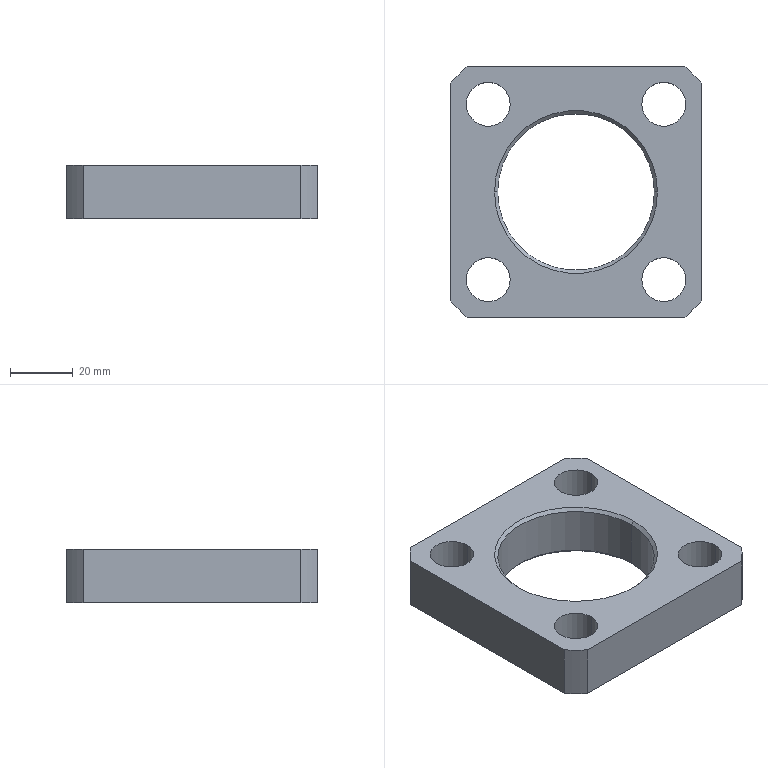Component | SolidWorks | Cylinder-1_Gland-1 | 1 solid | 24 faces | box 80 x 80 x 17 mm | volume 63907 mm3 | cylinder 14 | plane 6 | cone 4 | commonest cylinder face diameters 14 x8 106 x4 50 x2
STEP:
#1=CARTESIAN_POINT('',(-8.093,1.04,-7.612));
#2=VERTEX_POINT('',#1);
#3=CARTESIAN_POINT('',(-6.124,1.04,-7.612));
#4=VERTEX_POINT('',#3);
#5=CARTESIAN_POINT('',(-7.109,1.04,-7.612));
#6=DIRECTION('',(0.,-0.,-1.));
#7=DIRECTION('',(-1.,0.,0.));
#8=AXIS2_PLACEMENT_3D('',#5,#6,#7);
#9=CIRCLE('',#8,0.9843);
#10=EDGE_CURVE('',#2,#4,#9,.T.);
#11=ORIENTED_EDGE('',*,*,#10,.F.);
#12=CARTESIAN_POINT('',(-8.132,1.04,-7.652));
#13=VERTEX_POINT('',#12);
#14=CARTESIAN_POINT('',(-8.093,1.04,-7.612));
#15=DIRECTION('',(-0.7071,-0.,-0.7071));
#16=VECTOR('',#15,39.37);
#17=LINE('',#14,#16);
#18=EDGE_CURVE('',#2,#13,#17,.T.);
#19=ORIENTED_EDGE('',*,*,#18,.T.);
#20=CARTESIAN_POINT('',(-6.085,1.04,-7.652));
#21=VERTEX_POINT('',#20);
#22=CARTESIAN_POINT('',(-7.109,1.04,-7.652));
#23=DIRECTION('',(-0.,0.,1.));
#24=DIRECTION('',(-1.,0.,0.));
#25=AXIS2_PLACEMENT_3D('',#22,#23,#24);
#26=CIRCLE('',#25,1.024);
#27=EDGE_CURVE('',#21,#13,#26,.T.);
#28=ORIENTED_EDGE('',*,*,#27,.F.);
#29=CARTESIAN_POINT('',(-6.124,1.04,-7.612));
#30=DIRECTION('',(0.7071,-0.,-0.7071));
#31=VECTOR('',#30,39.37);
#32=LINE('',#29,#31);
#33=EDGE_CURVE('',#4,#21,#32,.T.);
#34=ORIENTED_EDGE('',*,*,#33,.F.);
#35=EDGE_LOOP('',(#11,#19,#28,#34));
#36=FACE_OUTER_BOUND('',#35,.T.);
#37=CARTESIAN_POINT('',(-7.109,1.04,-7.612));
#38=DIRECTION('',(0.,-0.,-1.));
#39=DIRECTION('',(1.,-0.,0.));
#40=AXIS2_PLACEMENT_3D('',#37,#38,#39);
#41=CONICAL_SURFACE('',#40,0.9843,0.7854);
#42=ADVANCED_FACE('',(#36),#41,.F.);
#43=CARTESIAN_POINT('',(-6.124,1.04,-7.022));
#44=VERTEX_POINT('',#43);
#45=CARTESIAN_POINT('',(-8.093,1.04,-7.022));
#46=VERTEX_POINT('',#45);
#47=CARTESIAN_POINT('',(-7.109,1.04,-7.022));
#48=DIRECTION('',(-0.,0.,1.));
#49=DIRECTION('',(-1.,0.,0.));
#50=AXIS2_PLACEMENT_3D('',#47,#48,#49);
#51=CIRCLE('',#50,0.9843);
#52=EDGE_CURVE('',#44,#46,#51,.T.);
#53=ORIENTED_EDGE('',*,*,#52,.F.);
#54=CARTESIAN_POINT('',(-6.085,1.04,-6.982));
#55=VERTEX_POINT('',#54);
#56=CARTESIAN_POINT('',(-6.085,1.04,-6.982));
#57=DIRECTION('',(0.7071,-0.,0.7071));
#58=VECTOR('',#57,39.37);
#59=LINE('',#56,#58);
#60=EDGE_CURVE('',#44,#55,#59,.T.);
#61=ORIENTED_EDGE('',*,*,#60,.T.);
#62=CARTESIAN_POINT('',(-8.132,1.04,-6.982));
#63=VERTEX_POINT('',#62);
#64=CARTESIAN_POINT('',(-7.109,1.04,-6.982));
#65=DIRECTION('',(0.,-0.,-1.));
#66=DIRECTION('',(-1.,0.,0.));
#67=AXIS2_PLACEMENT_3D('',#64,#65,#66);
#68=CIRCLE('',#67,1.024);
#69=EDGE_CURVE('',#63,#55,#68,.T.);
#70=ORIENTED_EDGE('',*,*,#69,.F.);
#71=CARTESIAN_POINT('',(-8.132,1.04,-6.982));
#72=DIRECTION('',(-0.7071,0.,0.7071));
#73=VECTOR('',#72,39.37);
#74=LINE('',#71,#73);
#75=EDGE_CURVE('',#46,#63,#74,.T.);
#76=ORIENTED_EDGE('',*,*,#75,.F.);
#77=EDGE_LOOP('',(#53,#61,#70,#76));
#78=FACE_OUTER_BOUND('',#77,.T.);
#79=CARTESIAN_POINT('',(-7.109,1.04,-6.982));
#80=DIRECTION('',(-0.,0.,1.));
#81=DIRECTION('',(-1.,0.,0.));
#82=AXIS2_PLACEMENT_3D('',#79,#80,#81);
#83=CONICAL_SURFACE('',#82,1.024,0.7854);
#84=ADVANCED_FACE('',(#78),#83,.F.);
#85=ORIENTED_EDGE('',*,*,#52,.T.);
#86=CARTESIAN_POINT('',(-8.093,1.04,-6.982));
#87=DIRECTION('',(0.,-0.,-1.));
#88=VECTOR('',#87,39.37);
#89=LINE('',#86,#88);
#90=EDGE_CURVE('',#46,#2,#89,.T.);
#91=ORIENTED_EDGE('',*,*,#90,.T.);
#92=ORIENTED_EDGE('',*,*,#10,.T.);
#93=CARTESIAN_POINT('',(-6.124,1.04,-6.982));
#94=DIRECTION('',(0.,-0.,-1.));
#95=VECTOR('',#94,39.37);
#96=LINE('',#93,#95);
#97=EDGE_CURVE('',#44,#4,#96,.T.);
#98=ORIENTED_EDGE('',*,*,#97,.F.);
#99=EDGE_LOOP('',(#85,#91,#92,#98));
#100=FACE_OUTER_BOUND('',#99,.T.);
#101=CARTESIAN_POINT('',(-7.109,1.04,-6.982));
#102=DIRECTION('',(0.,-0.,-1.));
#103=DIRECTION('',(1.,-0.,0.));
#104=AXIS2_PLACEMENT_3D('',#101,#102,#103);
#105=CYLINDRICAL_SURFACE('',#104,0.9843);
#106=ADVANCED_FACE('',(#100),#105,.F.);
#107=CARTESIAN_POINT('',(-8.486,2.142,-6.982));
#108=VERTEX_POINT('',#107);
#109=CARTESIAN_POINT('',(-7.935,2.142,-6.982));
#110=VERTEX_POINT('',#109);
#111=CARTESIAN_POINT('',(-8.211,2.142,-6.982));
#112=DIRECTION('',(0.,-0.,-1.));
#113=DIRECTION('',(-1.,0.,0.));
#114=AXIS2_PLACEMENT_3D('',#111,#112,#113);
#115=CIRCLE('',#114,0.2756);
#116=EDGE_CURVE('',#108,#110,#115,.T.);
#117=ORIENTED_EDGE('',*,*,#116,.F.);
#118=CARTESIAN_POINT('',(-8.486,2.142,-7.652));
#119=VERTEX_POINT('',#118);
#120=CARTESIAN_POINT('',(-8.486,2.142,-6.982));
#121=DIRECTION('',(0.,-0.,-1.));
#122=VECTOR('',#121,39.37);
#123=LINE('',#120,#122);
#124=EDGE_CURVE('',#108,#119,#123,.T.);
#125=ORIENTED_EDGE('',*,*,#124,.T.);
#126=CARTESIAN_POINT('',(-7.935,2.142,-7.652));
#127=VERTEX_POINT('',#126);
#128=CARTESIAN_POINT('',(-8.211,2.142,-7.652));
#129=DIRECTION('',(0.,-0.,-1.));
#130=DIRECTION('',(-1.,0.,0.));
#131=AXIS2_PLACEMENT_3D('',#128,#129,#130);
#132=CIRCLE('',#131,0.2756);
#133=EDGE_CURVE('',#119,#127,#132,.T.);
#134=ORIENTED_EDGE('',*,*,#133,.T.);
#135=CARTESIAN_POINT('',(-7.935,2.142,-6.982));
#136=DIRECTION('',(0.,-0.,-1.));
#137=VECTOR('',#136,39.37);
#138=LINE('',#135,#137);
#139=EDGE_CURVE('',#110,#127,#138,.T.);
#140=ORIENTED_EDGE('',*,*,#139,.F.);
#141=EDGE_LOOP('',(#117,#125,#134,#140));
#142=FACE_OUTER_BOUND('',#141,.T.);
#143=CARTESIAN_POINT('',(-8.211,2.142,-6.982));
#144=DIRECTION('',(0.,-0.,-1.));
#145=DIRECTION('',(1.,0.,0.));
#146=AXIS2_PLACEMENT_3D('',#143,#144,#145);
#147=CYLINDRICAL_SURFACE('',#146,0.2756);
#148=ADVANCED_FACE('',(#142),#147,.F.);
#149=CARTESIAN_POINT('',(-6.282,2.142,-6.982));
#150=VERTEX_POINT('',#149);
#151=CARTESIAN_POINT('',(-5.731,2.142,-6.982));
#152=VERTEX_POINT('',#151);
#153=CARTESIAN_POINT('',(-6.006,2.142,-6.982));
#154=DIRECTION('',(0.,-0.,-1.));
#155=DIRECTION('',(1.,0.,0.));
#156=AXIS2_PLACEMENT_3D('',#153,#154,#155);
#157=CIRCLE('',#156,0.2756);
#158=EDGE_CURVE('',#150,#152,#157,.T.);
#159=ORIENTED_EDGE('',*,*,#158,.F.);
#160=CARTESIAN_POINT('',(-6.282,2.142,-7.652));
#161=VERTEX_POINT('',#160);
#162=CARTESIAN_POINT('',(-6.282,2.142,-6.982));
#163=DIRECTION('',(0.,-0.,-1.));
#164=VECTOR('',#163,39.37);
#165=LINE('',#162,#164);
#166=EDGE_CURVE('',#150,#161,#165,.T.);
#167=ORIENTED_EDGE('',*,*,#166,.T.);
#168=CARTESIAN_POINT('',(-5.731,2.142,-7.652));
#169=VERTEX_POINT('',#168);
#170=CARTESIAN_POINT('',(-6.006,2.142,-7.652));
#171=DIRECTION('',(0.,-0.,-1.));
#172=DIRECTION('',(1.,0.,0.));
#173=AXIS2_PLACEMENT_3D('',#170,#171,#172);
#174=CIRCLE('',#173,0.2756);
#175=EDGE_CURVE('',#161,#169,#174,.T.);
#176=ORIENTED_EDGE('',*,*,#175,.T.);
#177=CARTESIAN_POINT('',(-5.731,2.142,-6.982));
#178=DIRECTION('',(0.,-0.,-1.));
#179=VECTOR('',#178,39.37);
#180=LINE('',#177,#179);
#181=EDGE_CURVE('',#152,#169,#180,.T.);
#182=ORIENTED_EDGE('',*,*,#181,.F.);
#183=EDGE_LOOP('',(#159,#167,#176,#182));
#184=FACE_OUTER_BOUND('',#183,.T.);
#185=CARTESIAN_POINT('',(-6.006,2.142,-6.982));
#186=DIRECTION('',(0.,-0.,-1.));
#187=DIRECTION('',(1.,0.,0.));
#188=AXIS2_PLACEMENT_3D('',#185,#186,#187);
#189=CYLINDRICAL_SURFACE('',#188,0.2756);
#190=ADVANCED_FACE('',(#184),#189,.F.);
#191=CARTESIAN_POINT('',(-6.282,-0.06252,-6.982));
#192=VERTEX_POINT('',#191);
#193=CARTESIAN_POINT('',(-5.731,-0.06252,-6.982));
#194=VERTEX_POINT('',#193);
#195=CARTESIAN_POINT('',(-6.006,-0.06252,-6.982));
#196=DIRECTION('',(0.,-0.,-1.));
#197=DIRECTION('',(-1.,0.,0.));
#198=AXIS2_PLACEMENT_3D('',#195,#196,#197);
#199=CIRCLE('',#198,0.2756);
#200=EDGE_CURVE('',#192,#194,#199,.T.);
#201=ORIENTED_EDGE('',*,*,#200,.F.);
#202=CARTESIAN_POINT('',(-6.282,-0.06252,-7.652));
#203=VERTEX_POINT('',#202);
#204=CARTESIAN_POINT('',(-6.282,-0.06252,-6.982));
#205=DIRECTION('',(0.,-0.,-1.));
#206=VECTOR('',#205,39.37);
#207=LINE('',#204,#206);
#208=EDGE_CURVE('',#192,#203,#207,.T.);
#209=ORIENTED_EDGE('',*,*,#208,.T.);
#210=CARTESIAN_POINT('',(-5.731,-0.06252,-7.652));
#211=VERTEX_POINT('',#210);
#212=CARTESIAN_POINT('',(-6.006,-0.06252,-7.652));
#213=DIRECTION('',(0.,-0.,-1.));
#214=DIRECTION('',(-1.,0.,0.));
#215=AXIS2_PLACEMENT_3D('',#212,#213,#214);
#216=CIRCLE('',#215,0.2756);
#217=EDGE_CURVE('',#203,#211,#216,.T.);
#218=ORIENTED_EDGE('',*,*,#217,.T.);
#219=CARTESIAN_POINT('',(-5.731,-0.06252,-6.982));
#220=DIRECTION('',(0.,-0.,-1.));
#221=VECTOR('',#220,39.37);
#222=LINE('',#219,#221);
#223=EDGE_CURVE('',#194,#211,#222,.T.);
#224=ORIENTED_EDGE('',*,*,#223,.F.);
#225=EDGE_LOOP('',(#201,#209,#218,#224));
#226=FACE_OUTER_BOUND('',#225,.T.);
#227=CARTESIAN_POINT('',(-6.006,-0.06252,-6.982));
#228=DIRECTION('',(0.,-0.,-1.));
#229=DIRECTION('',(1.,-0.,0.));
#230=AXIS2_PLACEMENT_3D('',#227,#228,#229);
#231=CYLINDRICAL_SURFACE('',#230,0.2756);
#232=ADVANCED_FACE('',(#226),#231,.F.);
#233=CARTESIAN_POINT('',(-8.486,-0.06252,-6.982));
#234=VERTEX_POINT('',#233);
#235=CARTESIAN_POINT('',(-7.935,-0.06252,-6.982));
#236=VERTEX_POINT('',#235);
#237=CARTESIAN_POINT('',(-8.211,-0.06252,-6.982));
#238=DIRECTION('',(0.,-0.,-1.));
#239=DIRECTION('',(1.,-0.,0.));
#240=AXIS2_PLACEMENT_3D('',#237,#238,#239);
#241=CIRCLE('',#240,0.2756);
#242=EDGE_CURVE('',#234,#236,#241,.T.);
#243=ORIENTED_EDGE('',*,*,#242,.F.);
#244=CARTESIAN_POINT('',(-8.486,-0.06252,-7.652));
#245=VERTEX_POINT('',#244);
#246=CARTESIAN_POINT('',(-8.486,-0.06252,-6.982));
#247=DIRECTION('',(0.,-0.,-1.));
#248=VECTOR('',#247,39.37);
#249=LINE('',#246,#248);
#250=EDGE_CURVE('',#234,#245,#249,.T.);
#251=ORIENTED_EDGE('',*,*,#250,.T.);
#252=CARTESIAN_POINT('',(-7.935,-0.06252,-7.652));
#253=VERTEX_POINT('',#252);
#254=CARTESIAN_POINT('',(-8.211,-0.06252,-7.652));
#255=DIRECTION('',(0.,-0.,-1.));
#256=DIRECTION('',(1.,-0.,0.));
#257=AXIS2_PLACEMENT_3D('',#254,#255,#256);
#258=CIRCLE('',#257,0.2756);
#259=EDGE_CURVE('',#245,#253,#258,.T.);
#260=ORIENTED_EDGE('',*,*,#259,.T.);
#261=CARTESIAN_POINT('',(-7.935,-0.06252,-6.982));
#262=DIRECTION('',(0.,-0.,-1.));
#263=VECTOR('',#262,39.37);
#264=LINE('',#261,#263);
#265=EDGE_CURVE('',#236,#253,#264,.T.);
#266=ORIENTED_EDGE('',*,*,#265,.F.);
#267=EDGE_LOOP('',(#243,#251,#260,#266));
#268=FACE_OUTER_BOUND('',#267,.T.);
#269=CARTESIAN_POINT('',(-8.211,-0.06252,-6.982));
#270=DIRECTION('',(0.,-0.,-1.));
#271=DIRECTION('',(1.,-0.,0.));
#272=AXIS2_PLACEMENT_3D('',#269,#270,#271);
#273=CYLINDRICAL_SURFACE('',#272,0.2756);
#274=ADVANCED_FACE('',(#268),#273,.F.);
#275=CARTESIAN_POINT('',(-8.683,-0.3291,-6.982));
#276=VERTEX_POINT('',#275);
#277=CARTESIAN_POINT('',(-8.683,2.409,-6.982));
#278=VERTEX_POINT('',#277);
#279=CARTESIAN_POINT('',(-8.683,2.615,-6.982));
#280=DIRECTION('',(0.,1.,-0.));
#281=VECTOR('',#280,39.37);
#282=LINE('',#279,#281);
#283=EDGE_CURVE('',#276,#278,#282,.T.);
#284=ORIENTED_EDGE('',*,*,#283,.T.);
#285=CARTESIAN_POINT('',(-8.683,2.409,-7.652));
#286=VERTEX_POINT('',#285);
#287=CARTESIAN_POINT('',(-8.683,2.409,-6.982));
#288=DIRECTION('',(0.,-0.,-1.));
#289=VECTOR('',#288,39.37);
#290=LINE('',#287,#289);
#291=EDGE_CURVE('',#278,#286,#290,.T.);
#292=ORIENTED_EDGE('',*,*,#291,.T.);
#293=CARTESIAN_POINT('',(-8.683,-0.3291,-7.652));
#294=VERTEX_POINT('',#293);
#295=CARTESIAN_POINT('',(-8.683,2.615,-7.652));
#296=DIRECTION('',(0.,1.,-0.));
#297=VECTOR('',#296,39.37);
#298=LINE('',#295,#297);
#299=EDGE_CURVE('',#294,#286,#298,.T.);
#300=ORIENTED_EDGE('',*,*,#299,.F.);
#301=CARTESIAN_POINT('',(-8.683,-0.3291,-6.982));
#302=DIRECTION('',(-0.,0.,1.));
#303=VECTOR('',#302,39.37);
#304=LINE('',#301,#303);
#305=EDGE_CURVE('',#294,#276,#304,.T.);
#306=ORIENTED_EDGE('',*,*,#305,.T.);
#307=EDGE_LOOP('',(#284,#292,#300,#306));
#308=FACE_OUTER_BOUND('',#307,.T.);
#309=CARTESIAN_POINT('',(-8.683,2.615,-6.982));
#310=DIRECTION('',(-1.,0.,-0.));
#311=DIRECTION('',(0.,-0.,-1.));
#312=AXIS2_PLACEMENT_3D('',#309,#310,#311);
#313=PLANE('',#312);
#314=ADVANCED_FACE('',(#308),#313,.T.);
#315=CARTESIAN_POINT('',(-5.74,-0.535,-6.982));
#316=VERTEX_POINT('',#315);
#317=CARTESIAN_POINT('',(-8.477,-0.535,-6.982));
#318=VERTEX_POINT('',#317);
#319=CARTESIAN_POINT('',(-8.683,-0.535,-6.982));
#320=DIRECTION('',(-1.,0.,-0.));
#321=VECTOR('',#320,39.37);
#322=LINE('',#319,#321);
#323=EDGE_CURVE('',#316,#318,#322,.T.);
#324=ORIENTED_EDGE('',*,*,#323,.T.);
#325=CARTESIAN_POINT('',(-8.477,-0.535,-7.652));
#326=VERTEX_POINT('',#325);
#327=CARTESIAN_POINT('',(-8.477,-0.535,-6.982));
#328=DIRECTION('',(0.,-0.,-1.));
#329=VECTOR('',#328,39.37);
#330=LINE('',#327,#329);
#331=EDGE_CURVE('',#318,#326,#330,.T.);
#332=ORIENTED_EDGE('',*,*,#331,.T.);
#333=CARTESIAN_POINT('',(-5.74,-0.535,-7.652));
#334=VERTEX_POINT('',#333);
#335=CARTESIAN_POINT('',(-8.683,-0.535,-7.652));
#336=DIRECTION('',(-1.,0.,-0.));
#337=VECTOR('',#336,39.37);
#338=LINE('',#335,#337);
#339=EDGE_CURVE('',#334,#326,#338,.T.);
#340=ORIENTED_EDGE('',*,*,#339,.F.);
#341=CARTESIAN_POINT('',(-5.74,-0.535,-6.982));
#342=DIRECTION('',(-0.,0.,1.));
#343=VECTOR('',#342,39.37);
#344=LINE('',#341,#343);
#345=EDGE_CURVE('',#334,#316,#344,.T.);
#346=ORIENTED_EDGE('',*,*,#345,.T.);
#347=EDGE_LOOP('',(#324,#332,#340,#346));
#348=FACE_OUTER_BOUND('',#347,.T.);
#349=CARTESIAN_POINT('',(-8.683,-0.535,-6.982));
#350=DIRECTION('',(-0.,-1.,0.));
#351=DIRECTION('',(0.,-0.,-1.));
#352=AXIS2_PLACEMENT_3D('',#349,#350,#351);
#353=PLANE('',#352);
#354=ADVANCED_FACE('',(#348),#353,.T.);
#355=CARTESIAN_POINT('',(-5.534,2.409,-6.982));
#356=VERTEX_POINT('',#355);
#357=CARTESIAN_POINT('',(-5.534,-0.3291,-6.982));
#358=VERTEX_POINT('',#357);
#359=CARTESIAN_POINT('',(-5.534,2.615,-6.982));
#360=DIRECTION('',(-0.,-1.,0.));
#361=VECTOR('',#360,39.37);
#362=LINE('',#359,#361);
#363=EDGE_CURVE('',#356,#358,#362,.T.);
#364=ORIENTED_EDGE('',*,*,#363,.T.);
#365=CARTESIAN_POINT('',(-5.534,-0.3291,-7.652));
#366=VERTEX_POINT('',#365);
#367=CARTESIAN_POINT('',(-5.534,-0.3291,-6.982));
#368=DIRECTION('',(0.,-0.,-1.));
#369=VECTOR('',#368,39.37);
#370=LINE('',#367,#369);
#371=EDGE_CURVE('',#358,#366,#370,.T.);
#372=ORIENTED_EDGE('',*,*,#371,.T.);
#373=CARTESIAN_POINT('',(-5.534,2.409,-7.652));
#374=VERTEX_POINT('',#373);
#375=CARTESIAN_POINT('',(-5.534,2.615,-7.652));
#376=DIRECTION('',(-0.,-1.,0.));
#377=VECTOR('',#376,39.37);
#378=LINE('',#375,#377);
#379=EDGE_CURVE('',#374,#366,#378,.T.);
#380=ORIENTED_EDGE('',*,*,#379,.F.);
#381=CARTESIAN_POINT('',(-5.534,2.409,-6.982));
#382=DIRECTION('',(-0.,0.,1.));
#383=VECTOR('',#382,39.37);
#384=LINE('',#381,#383);
#385=EDGE_CURVE('',#374,#356,#384,.T.);
#386=ORIENTED_EDGE('',*,*,#385,.T.);
#387=EDGE_LOOP('',(#364,#372,#380,#386));
#388=FACE_OUTER_BOUND('',#387,.T.);
#389=CARTESIAN_POINT('',(-5.534,2.615,-6.982));
#390=DIRECTION('',(1.,-0.,0.));
#391=DIRECTION('',(-0.,0.,1.));
#392=AXIS2_PLACEMENT_3D('',#389,#390,#391);
#393=PLANE('',#392);
#394=ADVANCED_FACE('',(#388),#393,.T.);
#395=CARTESIAN_POINT('',(-8.477,2.615,-6.982));
#396=VERTEX_POINT('',#395);
#397=CARTESIAN_POINT('',(-5.74,2.615,-6.982));
#398=VERTEX_POINT('',#397);
#399=CARTESIAN_POINT('',(-8.683,2.615,-6.982));
#400=DIRECTION('',(1.,-0.,0.));
#401=VECTOR('',#400,39.37);
#402=LINE('',#399,#401);
#403=EDGE_CURVE('',#396,#398,#402,.T.);
#404=ORIENTED_EDGE('',*,*,#403,.T.);
#405=CARTESIAN_POINT('',(-5.74,2.615,-7.652));
#406=VERTEX_POINT('',#405);
#407=CARTESIAN_POINT('',(-5.74,2.615,-6.982));
#408=DIRECTION('',(0.,-0.,-1.));
#409=VECTOR('',#408,39.37);
#410=LINE('',#407,#409);
#411=EDGE_CURVE('',#398,#406,#410,.T.);
#412=ORIENTED_EDGE('',*,*,#411,.T.);
#413=CARTESIAN_POINT('',(-8.477,2.615,-7.652));
#414=VERTEX_POINT('',#413);
#415=CARTESIAN_POINT('',(-8.683,2.615,-7.652));
#416=DIRECTION('',(1.,-0.,0.));
#417=VECTOR('',#416,39.37);
#418=LINE('',#415,#417);
#419=EDGE_CURVE('',#414,#406,#418,.T.);
#420=ORIENTED_EDGE('',*,*,#419,.F.);
#421=CARTESIAN_POINT('',(-8.477,2.615,-6.982));
#422=DIRECTION('',(-0.,0.,1.));
#423=VECTOR('',#422,39.37);
#424=LINE('',#421,#423);
#425=EDGE_CURVE('',#414,#396,#424,.T.);
#426=ORIENTED_EDGE('',*,*,#425,.T.);
#427=EDGE_LOOP('',(#404,#412,#420,#426));
#428=FACE_OUTER_BOUND('',#427,.T.);
#429=CARTESIAN_POINT('',(-8.683,2.615,-6.982));
#430=DIRECTION('',(0.,1.,-0.));
#431=DIRECTION('',(-0.,0.,1.));
#432=AXIS2_PLACEMENT_3D('',#429,#430,#431);
#433=PLANE('',#432);
#434=ADVANCED_FACE('',(#428),#433,.T.);
#435=ORIENTED_EDGE('',*,*,#69,.T.);
#436=CARTESIAN_POINT('',(-7.109,1.04,-6.982));
#437=DIRECTION('',(0.,-0.,-1.));
#438=DIRECTION('',(-1.,0.,0.));
#439=AXIS2_PLACEMENT_3D('',#436,#437,#438);
#440=CIRCLE('',#439,1.024);
#441=EDGE_CURVE('',#55,#63,#440,.T.);
#442=ORIENTED_EDGE('',*,*,#441,.T.);
#443=EDGE_LOOP('',(#435,#442));
#444=FACE_BOUND('',#443,.T.);
#445=CARTESIAN_POINT('',(-8.211,2.142,-6.982));
#446=DIRECTION('',(0.,-0.,-1.));
#447=DIRECTION('',(-1.,0.,0.));
#448=AXIS2_PLACEMENT_3D('',#445,#446,#447);
#449=CIRCLE('',#448,0.2756);
#450=EDGE_CURVE('',#110,#108,#449,.T.);
#451=ORIENTED_EDGE('',*,*,#450,.T.);
#452=ORIENTED_EDGE('',*,*,#116,.T.);
#453=EDGE_LOOP('',(#451,#452));
#454=FACE_BOUND('',#453,.T.);
#455=CARTESIAN_POINT('',(-6.006,2.142,-6.982));
#456=DIRECTION('',(0.,-0.,-1.));
#457=DIRECTION('',(1.,0.,0.));
#458=AXIS2_PLACEMENT_3D('',#455,#456,#457);
#459=CIRCLE('',#458,0.2756);
#460=EDGE_CURVE('',#152,#150,#459,.T.);
#461=ORIENTED_EDGE('',*,*,#460,.T.);
#462=ORIENTED_EDGE('',*,*,#158,.T.);
#463=EDGE_LOOP('',(#461,#462));
#464=FACE_BOUND('',#463,.T.);
#465=CARTESIAN_POINT('',(-6.006,-0.06252,-6.982));
#466=DIRECTION('',(0.,-0.,-1.));
#467=DIRECTION('',(-1.,0.,0.));
#468=AXIS2_PLACEMENT_3D('',#465,#466,#467);
#469=CIRCLE('',#468,0.2756);
#470=EDGE_CURVE('',#194,#192,#469,.T.);
#471=ORIENTED_EDGE('',*,*,#470,.T.);
#472=ORIENTED_EDGE('',*,*,#200,.T.);
#473=EDGE_LOOP('',(#471,#472));
#474=FACE_BOUND('',#473,.T.);
#475=CARTESIAN_POINT('',(-8.211,-0.06252,-6.982));
#476=DIRECTION('',(0.,-0.,-1.));
#477=DIRECTION('',(1.,-0.,0.));
#478=AXIS2_PLACEMENT_3D('',#475,#476,#477);
#479=CIRCLE('',#478,0.2756);
#480=EDGE_CURVE('',#236,#234,#479,.T.);
#481=ORIENTED_EDGE('',*,*,#480,.T.);
#482=ORIENTED_EDGE('',*,*,#242,.T.);
#483=EDGE_LOOP('',(#481,#482));
#484=FACE_BOUND('',#483,.T.);
#485=ORIENTED_EDGE('',*,*,#283,.F.);
#486=CARTESIAN_POINT('',(-7.109,1.04,-6.982));
#487=DIRECTION('',(0.,-0.,-1.));
#488=DIRECTION('',(1.,-0.,0.));
#489=AXIS2_PLACEMENT_3D('',#486,#487,#488);
#490=CIRCLE('',#489,2.087);
#491=EDGE_CURVE('',#318,#276,#490,.T.);
#492=ORIENTED_EDGE('',*,*,#491,.F.);
#493=ORIENTED_EDGE('',*,*,#323,.F.);
#494=CARTESIAN_POINT('',(-7.109,1.04,-6.982));
#495=DIRECTION('',(0.,-0.,-1.));
#496=DIRECTION('',(1.,-0.,0.));
#497=AXIS2_PLACEMENT_3D('',#494,#495,#496);
#498=CIRCLE('',#497,2.087);
#499=EDGE_CURVE('',#358,#316,#498,.T.);
#500=ORIENTED_EDGE('',*,*,#499,.F.);
#501=ORIENTED_EDGE('',*,*,#363,.F.);
#502=CARTESIAN_POINT('',(-7.109,1.04,-6.982));
#503=DIRECTION('',(0.,-0.,-1.));
#504=DIRECTION('',(1.,-0.,0.));
#505=AXIS2_PLACEMENT_3D('',#502,#503,#504);
#506=CIRCLE('',#505,2.087);
#507=EDGE_CURVE('',#398,#356,#506,.T.);
#508=ORIENTED_EDGE('',*,*,#507,.F.);
#509=ORIENTED_EDGE('',*,*,#403,.F.);
#510=CARTESIAN_POINT('',(-7.109,1.04,-6.982));
#511=DIRECTION('',(0.,-0.,-1.));
#512=DIRECTION('',(1.,-0.,0.));
#513=AXIS2_PLACEMENT_3D('',#510,#511,#512);
#514=CIRCLE('',#513,2.087);
#515=EDGE_CURVE('',#278,#396,#514,.T.);
#516=ORIENTED_EDGE('',*,*,#515,.F.);
#517=EDGE_LOOP('',(#485,#492,#493,#500,#501,#508,#509,#516));
#518=FACE_OUTER_BOUND('',#517,.T.);
#519=CARTESIAN_POINT('',(-8.683,2.615,-6.982));
#520=DIRECTION('',(-0.,0.,1.));
#521=DIRECTION('',(-1.,0.,-0.));
#522=AXIS2_PLACEMENT_3D('',#519,#520,#521);
#523=PLANE('',#522);
#524=ADVANCED_FACE('',(#444,#454,#464,#474,#484,#518),#523,.T.);
#525=ORIENTED_EDGE('',*,*,#27,.T.);
#526=CARTESIAN_POINT('',(-7.109,1.04,-7.652));
#527=DIRECTION('',(-0.,0.,1.));
#528=DIRECTION('',(-1.,0.,0.));
#529=AXIS2_PLACEMENT_3D('',#526,#527,#528);
#530=CIRCLE('',#529,1.024);
#531=EDGE_CURVE('',#13,#21,#530,.T.);
#532=ORIENTED_EDGE('',*,*,#531,.T.);
#533=EDGE_LOOP('',(#525,#532));
#534=FACE_BOUND('',#533,.T.);
#535=CARTESIAN_POINT('',(-8.211,2.142,-7.652));
#536=DIRECTION('',(0.,-0.,-1.));
#537=DIRECTION('',(-1.,0.,0.));
#538=AXIS2_PLACEMENT_3D('',#535,#536,#537);
#539=CIRCLE('',#538,0.2756);
#540=EDGE_CURVE('',#127,#119,#539,.T.);
#541=ORIENTED_EDGE('',*,*,#540,.F.);
#542=ORIENTED_EDGE('',*,*,#133,.F.);
#543=EDGE_LOOP('',(#541,#542));
#544=FACE_BOUND('',#543,.T.);
#545=CARTESIAN_POINT('',(-6.006,2.142,-7.652));
#546=DIRECTION('',(0.,-0.,-1.));
#547=DIRECTION('',(1.,0.,0.));
#548=AXIS2_PLACEMENT_3D('',#545,#546,#547);
#549=CIRCLE('',#548,0.2756);
#550=EDGE_CURVE('',#169,#161,#549,.T.);
#551=ORIENTED_EDGE('',*,*,#550,.F.);
#552=ORIENTED_EDGE('',*,*,#175,.F.);
#553=EDGE_LOOP('',(#551,#552));
#554=FACE_BOUND('',#553,.T.);
#555=CARTESIAN_POINT('',(-6.006,-0.06252,-7.652));
#556=DIRECTION('',(0.,-0.,-1.));
#557=DIRECTION('',(-1.,0.,0.));
#558=AXIS2_PLACEMENT_3D('',#555,#556,#557);
#559=CIRCLE('',#558,0.2756);
#560=EDGE_CURVE('',#211,#203,#559,.T.);
#561=ORIENTED_EDGE('',*,*,#560,.F.);
#562=ORIENTED_EDGE('',*,*,#217,.F.);
#563=EDGE_LOOP('',(#561,#562));
#564=FACE_BOUND('',#563,.T.);
#565=CARTESIAN_POINT('',(-8.211,-0.06252,-7.652));
#566=DIRECTION('',(0.,-0.,-1.));
#567=DIRECTION('',(1.,-0.,0.));
#568=AXIS2_PLACEMENT_3D('',#565,#566,#567);
#569=CIRCLE('',#568,0.2756);
#570=EDGE_CURVE('',#253,#245,#569,.T.);
#571=ORIENTED_EDGE('',*,*,#570,.F.);
#572=ORIENTED_EDGE('',*,*,#259,.F.);
#573=EDGE_LOOP('',(#571,#572));
#574=FACE_BOUND('',#573,.T.);
#575=CARTESIAN_POINT('',(-7.109,1.04,-7.652));
#576=DIRECTION('',(-0.,0.,1.));
#577=DIRECTION('',(-1.,0.,0.));
#578=AXIS2_PLACEMENT_3D('',#575,#576,#577);
#579=CIRCLE('',#578,2.087);
#580=EDGE_CURVE('',#294,#326,#579,.T.);
#581=ORIENTED_EDGE('',*,*,#580,.F.);
#582=ORIENTED_EDGE('',*,*,#299,.T.);
#583=CARTESIAN_POINT('',(-7.109,1.04,-7.652));
#584=DIRECTION('',(-0.,0.,1.));
#585=DIRECTION('',(-1.,0.,0.));
#586=AXIS2_PLACEMENT_3D('',#583,#584,#585);
#587=CIRCLE('',#586,2.087);
#588=EDGE_CURVE('',#414,#286,#587,.T.);
#589=ORIENTED_EDGE('',*,*,#588,.F.);
#590=ORIENTED_EDGE('',*,*,#419,.T.);
#591=CARTESIAN_POINT('',(-7.109,1.04,-7.652));
#592=DIRECTION('',(-0.,0.,1.));
#593=DIRECTION('',(-1.,0.,0.));
#594=AXIS2_PLACEMENT_3D('',#591,#592,#593);
#595=CIRCLE('',#594,2.087);
#596=EDGE_CURVE('',#374,#406,#595,.T.);
#597=ORIENTED_EDGE('',*,*,#596,.F.);
#598=ORIENTED_EDGE('',*,*,#379,.T.);
#599=CARTESIAN_POINT('',(-7.109,1.04,-7.652));
#600=DIRECTION('',(0.,-0.,-1.));
#601=DIRECTION('',(1.,-0.,0.));
#602=AXIS2_PLACEMENT_3D('',#599,#600,#601);
#603=CIRCLE('',#602,2.087);
#604=EDGE_CURVE('',#366,#334,#603,.T.);
#605=ORIENTED_EDGE('',*,*,#604,.T.);
#606=ORIENTED_EDGE('',*,*,#339,.T.);
#607=EDGE_LOOP('',(#581,#582,#589,#590,#597,#598,#605,#606));
#608=FACE_OUTER_BOUND('',#607,.T.);
#609=CARTESIAN_POINT('',(-8.683,2.615,-7.652));
#610=DIRECTION('',(-0.,0.,1.));
#611=DIRECTION('',(-1.,0.,-0.));
#612=AXIS2_PLACEMENT_3D('',#609,#610,#611);
#613=PLANE('',#612);
#614=ADVANCED_FACE('',(#534,#544,#554,#564,#574,#608),#613,.F.);
#615=ORIENTED_EDGE('',*,*,#250,.F.);
#616=ORIENTED_EDGE('',*,*,#480,.F.);
#617=ORIENTED_EDGE('',*,*,#265,.T.);
#618=ORIENTED_EDGE('',*,*,#570,.T.);
#619=EDGE_LOOP('',(#615,#616,#617,#618));
#620=FACE_OUTER_BOUND('',#619,.T.);
#621=CARTESIAN_POINT('',(-8.211,-0.06252,-6.982));
#622=DIRECTION('',(0.,-0.,-1.));
#623=DIRECTION('',(1.,-0.,0.));
#624=AXIS2_PLACEMENT_3D('',#621,#622,#623);
#625=CYLINDRICAL_SURFACE('',#624,0.2756);
#626=ADVANCED_FACE('',(#620),#625,.F.);
#627=ORIENTED_EDGE('',*,*,#208,.F.);
#628=ORIENTED_EDGE('',*,*,#470,.F.);
#629=ORIENTED_EDGE('',*,*,#223,.T.);
#630=ORIENTED_EDGE('',*,*,#560,.T.);
#631=EDGE_LOOP('',(#627,#628,#629,#630));
#632=FACE_OUTER_BOUND('',#631,.T.);
#633=CARTESIAN_POINT('',(-6.006,-0.06252,-6.982));
#634=DIRECTION('',(0.,-0.,-1.));
#635=DIRECTION('',(1.,-0.,0.));
#636=AXIS2_PLACEMENT_3D('',#633,#634,#635);
#637=CYLINDRICAL_SURFACE('',#636,0.2756);
#638=ADVANCED_FACE('',(#632),#637,.F.);
#639=ORIENTED_EDGE('',*,*,#166,.F.);
#640=ORIENTED_EDGE('',*,*,#460,.F.);
#641=ORIENTED_EDGE('',*,*,#181,.T.);
#642=ORIENTED_EDGE('',*,*,#550,.T.);
#643=EDGE_LOOP('',(#639,#640,#641,#642));
#644=FACE_OUTER_BOUND('',#643,.T.);
#645=CARTESIAN_POINT('',(-6.006,2.142,-6.982));
#646=DIRECTION('',(0.,-0.,-1.));
#647=DIRECTION('',(1.,0.,0.));
#648=AXIS2_PLACEMENT_3D('',#645,#646,#647);
#649=CYLINDRICAL_SURFACE('',#648,0.2756);
#650=ADVANCED_FACE('',(#644),#649,.F.);
#651=ORIENTED_EDGE('',*,*,#124,.F.);
#652=ORIENTED_EDGE('',*,*,#450,.F.);
#653=ORIENTED_EDGE('',*,*,#139,.T.);
#654=ORIENTED_EDGE('',*,*,#540,.T.);
#655=EDGE_LOOP('',(#651,#652,#653,#654));
#656=FACE_OUTER_BOUND('',#655,.T.);
#657=CARTESIAN_POINT('',(-8.211,2.142,-6.982));
#658=DIRECTION('',(0.,-0.,-1.));
#659=DIRECTION('',(1.,0.,0.));
#660=AXIS2_PLACEMENT_3D('',#657,#658,#659);
#661=CYLINDRICAL_SURFACE('',#660,0.2756);
#662=ADVANCED_FACE('',(#656),#661,.F.);
#663=ORIENTED_EDGE('',*,*,#90,.F.);
#664=CARTESIAN_POINT('',(-7.109,1.04,-7.022));
#665=DIRECTION('',(-0.,0.,1.));
#666=DIRECTION('',(-1.,0.,0.));
#667=AXIS2_PLACEMENT_3D('',#664,#665,#666);
#668=CIRCLE('',#667,0.9843);
#669=EDGE_CURVE('',#46,#44,#668,.T.);
#670=ORIENTED_EDGE('',*,*,#669,.T.);
#671=ORIENTED_EDGE('',*,*,#97,.T.);
#672=CARTESIAN_POINT('',(-7.109,1.04,-7.612));
#673=DIRECTION('',(0.,-0.,-1.));
#674=DIRECTION('',(-1.,0.,0.));
#675=AXIS2_PLACEMENT_3D('',#672,#673,#674);
#676=CIRCLE('',#675,0.9843);
#677=EDGE_CURVE('',#4,#2,#676,.T.);
#678=ORIENTED_EDGE('',*,*,#677,.T.);
#679=EDGE_LOOP('',(#663,#670,#671,#678));
#680=FACE_OUTER_BOUND('',#679,.T.);
#681=CARTESIAN_POINT('',(-7.109,1.04,-6.982));
#682=DIRECTION('',(0.,-0.,-1.));
#683=DIRECTION('',(1.,-0.,0.));
#684=AXIS2_PLACEMENT_3D('',#681,#682,#683);
#685=CYLINDRICAL_SURFACE('',#684,0.9843);
#686=ADVANCED_FACE('',(#680),#685,.F.);
#687=ORIENTED_EDGE('',*,*,#515,.T.);
#688=ORIENTED_EDGE('',*,*,#425,.F.);
#689=ORIENTED_EDGE('',*,*,#588,.T.);
#690=ORIENTED_EDGE('',*,*,#291,.F.);
#691=EDGE_LOOP('',(#687,#688,#689,#690));
#692=FACE_OUTER_BOUND('',#691,.T.);
#693=CARTESIAN_POINT('',(-7.109,1.04,-6.982));
#694=DIRECTION('',(0.,-0.,-1.));
#695=DIRECTION('',(1.,-0.,0.));
#696=AXIS2_PLACEMENT_3D('',#693,#694,#695);
#697=CYLINDRICAL_SURFACE('',#696,2.087);
#698=ADVANCED_FACE('',(#692),#697,.T.);
#699=ORIENTED_EDGE('',*,*,#596,.T.);
#700=ORIENTED_EDGE('',*,*,#411,.F.);
#701=ORIENTED_EDGE('',*,*,#507,.T.);
#702=ORIENTED_EDGE('',*,*,#385,.F.);
#703=EDGE_LOOP('',(#699,#700,#701,#702));
#704=FACE_OUTER_BOUND('',#703,.T.);
#705=CARTESIAN_POINT('',(-7.109,1.04,-6.982));
#706=DIRECTION('',(0.,-0.,-1.));
#707=DIRECTION('',(1.,-0.,0.));
#708=AXIS2_PLACEMENT_3D('',#705,#706,#707);
#709=CYLINDRICAL_SURFACE('',#708,2.087);
#710=ADVANCED_FACE('',(#704),#709,.T.);
#711=ORIENTED_EDGE('',*,*,#604,.F.);
#712=ORIENTED_EDGE('',*,*,#371,.F.);
#713=ORIENTED_EDGE('',*,*,#499,.T.);
#714=ORIENTED_EDGE('',*,*,#345,.F.);
#715=EDGE_LOOP('',(#711,#712,#713,#714));
#716=FACE_OUTER_BOUND('',#715,.T.);
#717=CARTESIAN_POINT('',(-7.109,1.04,-6.982));
#718=DIRECTION('',(0.,-0.,-1.));
#719=DIRECTION('',(1.,-0.,0.));
#720=AXIS2_PLACEMENT_3D('',#717,#718,#719);
#721=CYLINDRICAL_SURFACE('',#720,2.087);
#722=ADVANCED_FACE('',(#716),#721,.T.);
#723=ORIENTED_EDGE('',*,*,#580,.T.);
#724=ORIENTED_EDGE('',*,*,#331,.F.);
#725=ORIENTED_EDGE('',*,*,#491,.T.);
#726=ORIENTED_EDGE('',*,*,#305,.F.);
#727=EDGE_LOOP('',(#723,#724,#725,#726));
#728=FACE_OUTER_BOUND('',#727,.T.);
#729=CARTESIAN_POINT('',(-7.109,1.04,-6.982));
#730=DIRECTION('',(0.,-0.,-1.));
#731=DIRECTION('',(1.,-0.,0.));
#732=AXIS2_PLACEMENT_3D('',#729,#730,#731);
#733=CYLINDRICAL_SURFACE('',#732,2.087);
#734=ADVANCED_FACE('',(#728),#733,.T.);
#735=ORIENTED_EDGE('',*,*,#60,.F.);
#736=ORIENTED_EDGE('',*,*,#669,.F.);
#737=ORIENTED_EDGE('',*,*,#75,.T.);
#738=ORIENTED_EDGE('',*,*,#441,.F.);
#739=EDGE_LOOP('',(#735,#736,#737,#738));
#740=FACE_OUTER_BOUND('',#739,.T.);
#741=CARTESIAN_POINT('',(-7.109,1.04,-6.982));
#742=DIRECTION('',(-0.,0.,1.));
#743=DIRECTION('',(-1.,0.,0.));
#744=AXIS2_PLACEMENT_3D('',#741,#742,#743);
#745=CONICAL_SURFACE('',#744,1.024,0.7854);
#746=ADVANCED_FACE('',(#740),#745,.F.);
#747=ORIENTED_EDGE('',*,*,#18,.F.);
#748=ORIENTED_EDGE('',*,*,#677,.F.);
#749=ORIENTED_EDGE('',*,*,#33,.T.);
#750=ORIENTED_EDGE('',*,*,#531,.F.);
#751=EDGE_LOOP('',(#747,#748,#749,#750));
#752=FACE_OUTER_BOUND('',#751,.T.);
#753=CARTESIAN_POINT('',(-7.109,1.04,-7.612));
#754=DIRECTION('',(0.,-0.,-1.));
#755=DIRECTION('',(1.,-0.,0.));
#756=AXIS2_PLACEMENT_3D('',#753,#754,#755);
#757=CONICAL_SURFACE('',#756,0.9843,0.7854);
#758=ADVANCED_FACE('',(#752),#757,.F.);
#759=CLOSED_SHELL('',(#42,#84,#106,#148,#190,#232,#274,#314,#354,#394,#434,#524,#614,#626,#638,#650,#662,#686,#698,#710,#722,#734,#746,#758));
#760=MANIFOLD_SOLID_BREP('',#759);
#761=CARTESIAN_POINT('',(0.,0.,0.));
#762=DIRECTION('',(0.,0.,1.));
#763=DIRECTION('',(1.,0.,0.));
#764=AXIS2_PLACEMENT_3D('',#761,#762,#763);
#765=(LENGTH_UNIT()NAMED_UNIT(*)SI_UNIT($,.METRE.));
#766=LENGTH_MEASURE_WITH_UNIT(LENGTH_MEASURE(0.0254),#765);
#767=DIMENSIONAL_EXPONENTS(1.,0.,0.,0.,0.,0.,0.);
#768=(CONVERSION_BASED_UNIT('',#766)LENGTH_UNIT()NAMED_UNIT(#767));
#769=UNCERTAINTY_MEASURE_WITH_UNIT(LENGTH_MEASURE(0.00001),#768,'','');
#770=(NAMED_UNIT(*)PLANE_ANGLE_UNIT()SI_UNIT($,.RADIAN.));
#771=(NAMED_UNIT(*)SI_UNIT($,.STERADIAN.)SOLID_ANGLE_UNIT());
#772=(GEOMETRIC_REPRESENTATION_CONTEXT(3)GLOBAL_UNCERTAINTY_ASSIGNED_CONTEXT((#769))GLOBAL_UNIT_ASSIGNED_CONTEXT((#768,#770,#771))REPRESENTATION_CONTEXT('',''));
#773=ADVANCED_BREP_SHAPE_REPRESENTATION('',(#760,#764),#772);
#774=COLOUR_RGB('',0.7922,0.8196,0.9333);
#775=FILL_AREA_STYLE_COLOUR('',#774);
#776=FILL_AREA_STYLE('',(#775));
#777=SURFACE_STYLE_FILL_AREA(#776);
#778=SURFACE_SIDE_STYLE('',(#777));
#779=SURFACE_STYLE_USAGE(.BOTH.,#778);
#780=PRESENTATION_STYLE_ASSIGNMENT((#779));
#781=STYLED_ITEM('',(#780),#760);
#782=(LENGTH_UNIT()NAMED_UNIT(*)SI_UNIT($,.METRE.));
#783=LENGTH_MEASURE_WITH_UNIT(LENGTH_MEASURE(0.0254),#782);
#784=DIMENSIONAL_EXPONENTS(1.,0.,0.,0.,0.,0.,0.);
#785=(CONVERSION_BASED_UNIT('',#783)LENGTH_UNIT()NAMED_UNIT(#784));
#786=UNCERTAINTY_MEASURE_WITH_UNIT(LENGTH_MEASURE(0.00001),#785,'','');
#787=(NAMED_UNIT(*)PLANE_ANGLE_UNIT()SI_UNIT($,.RADIAN.));
#788=(NAMED_UNIT(*)SI_UNIT($,.STERADIAN.)SOLID_ANGLE_UNIT());
#789=(GEOMETRIC_REPRESENTATION_CONTEXT(3)GLOBAL_UNCERTAINTY_ASSIGNED_CONTEXT((#786))GLOBAL_UNIT_ASSIGNED_CONTEXT((#785,#787,#788))REPRESENTATION_CONTEXT('',''));
#790=MECHANICAL_DESIGN_GEOMETRIC_PRESENTATION_REPRESENTATION('',(#781),#789);
#791=PRESENTATION_LAYER_ASSIGNMENT('','',(#781));